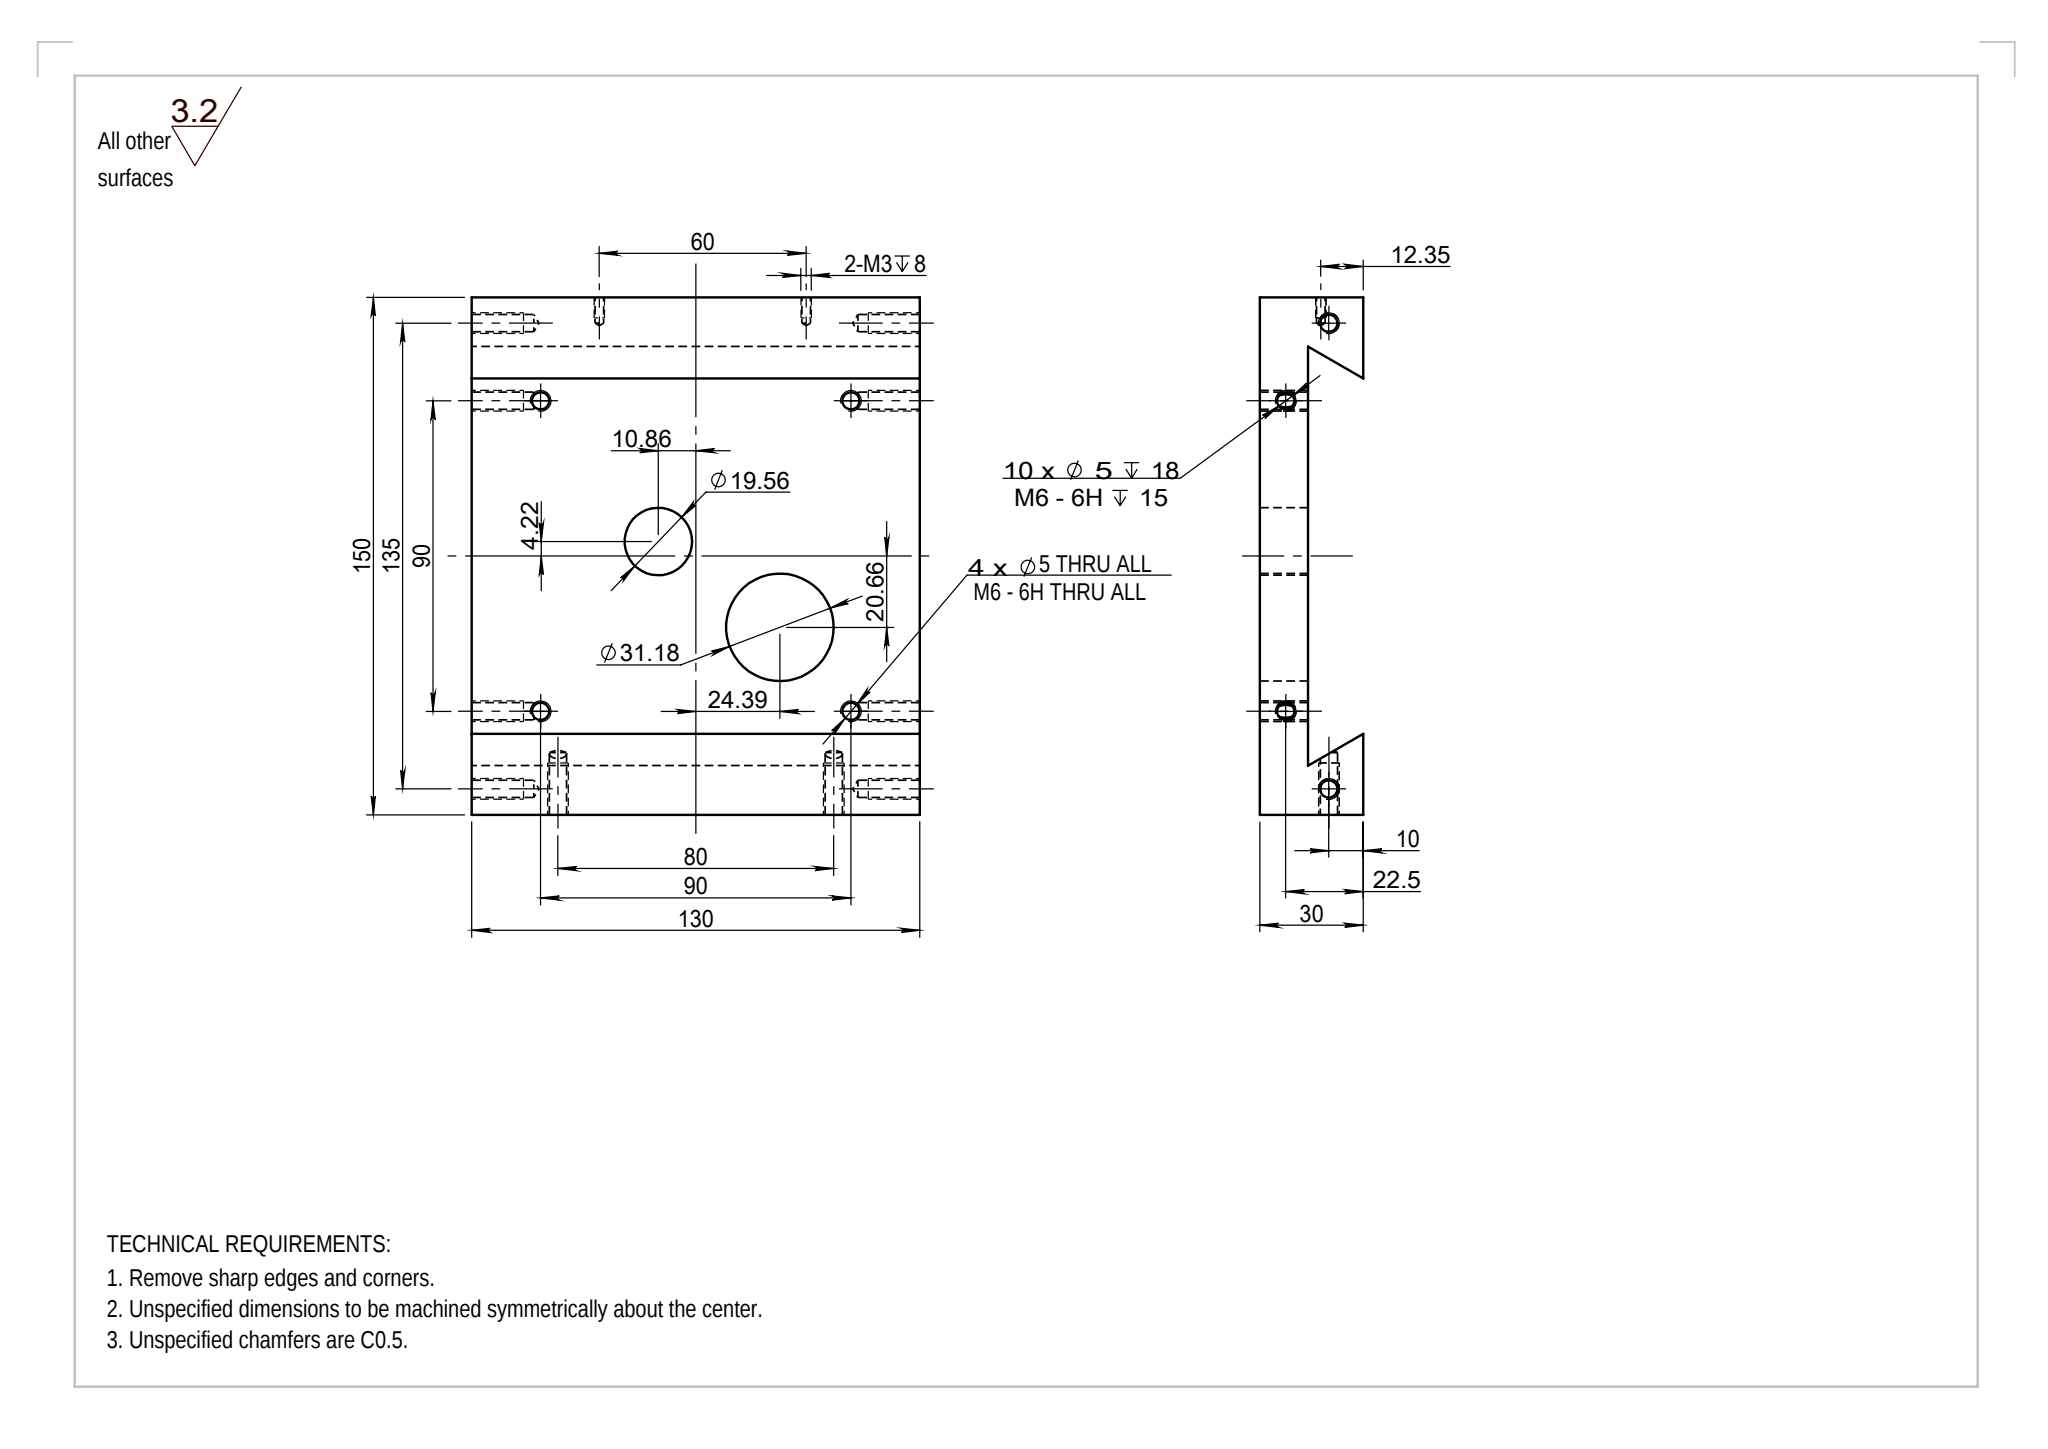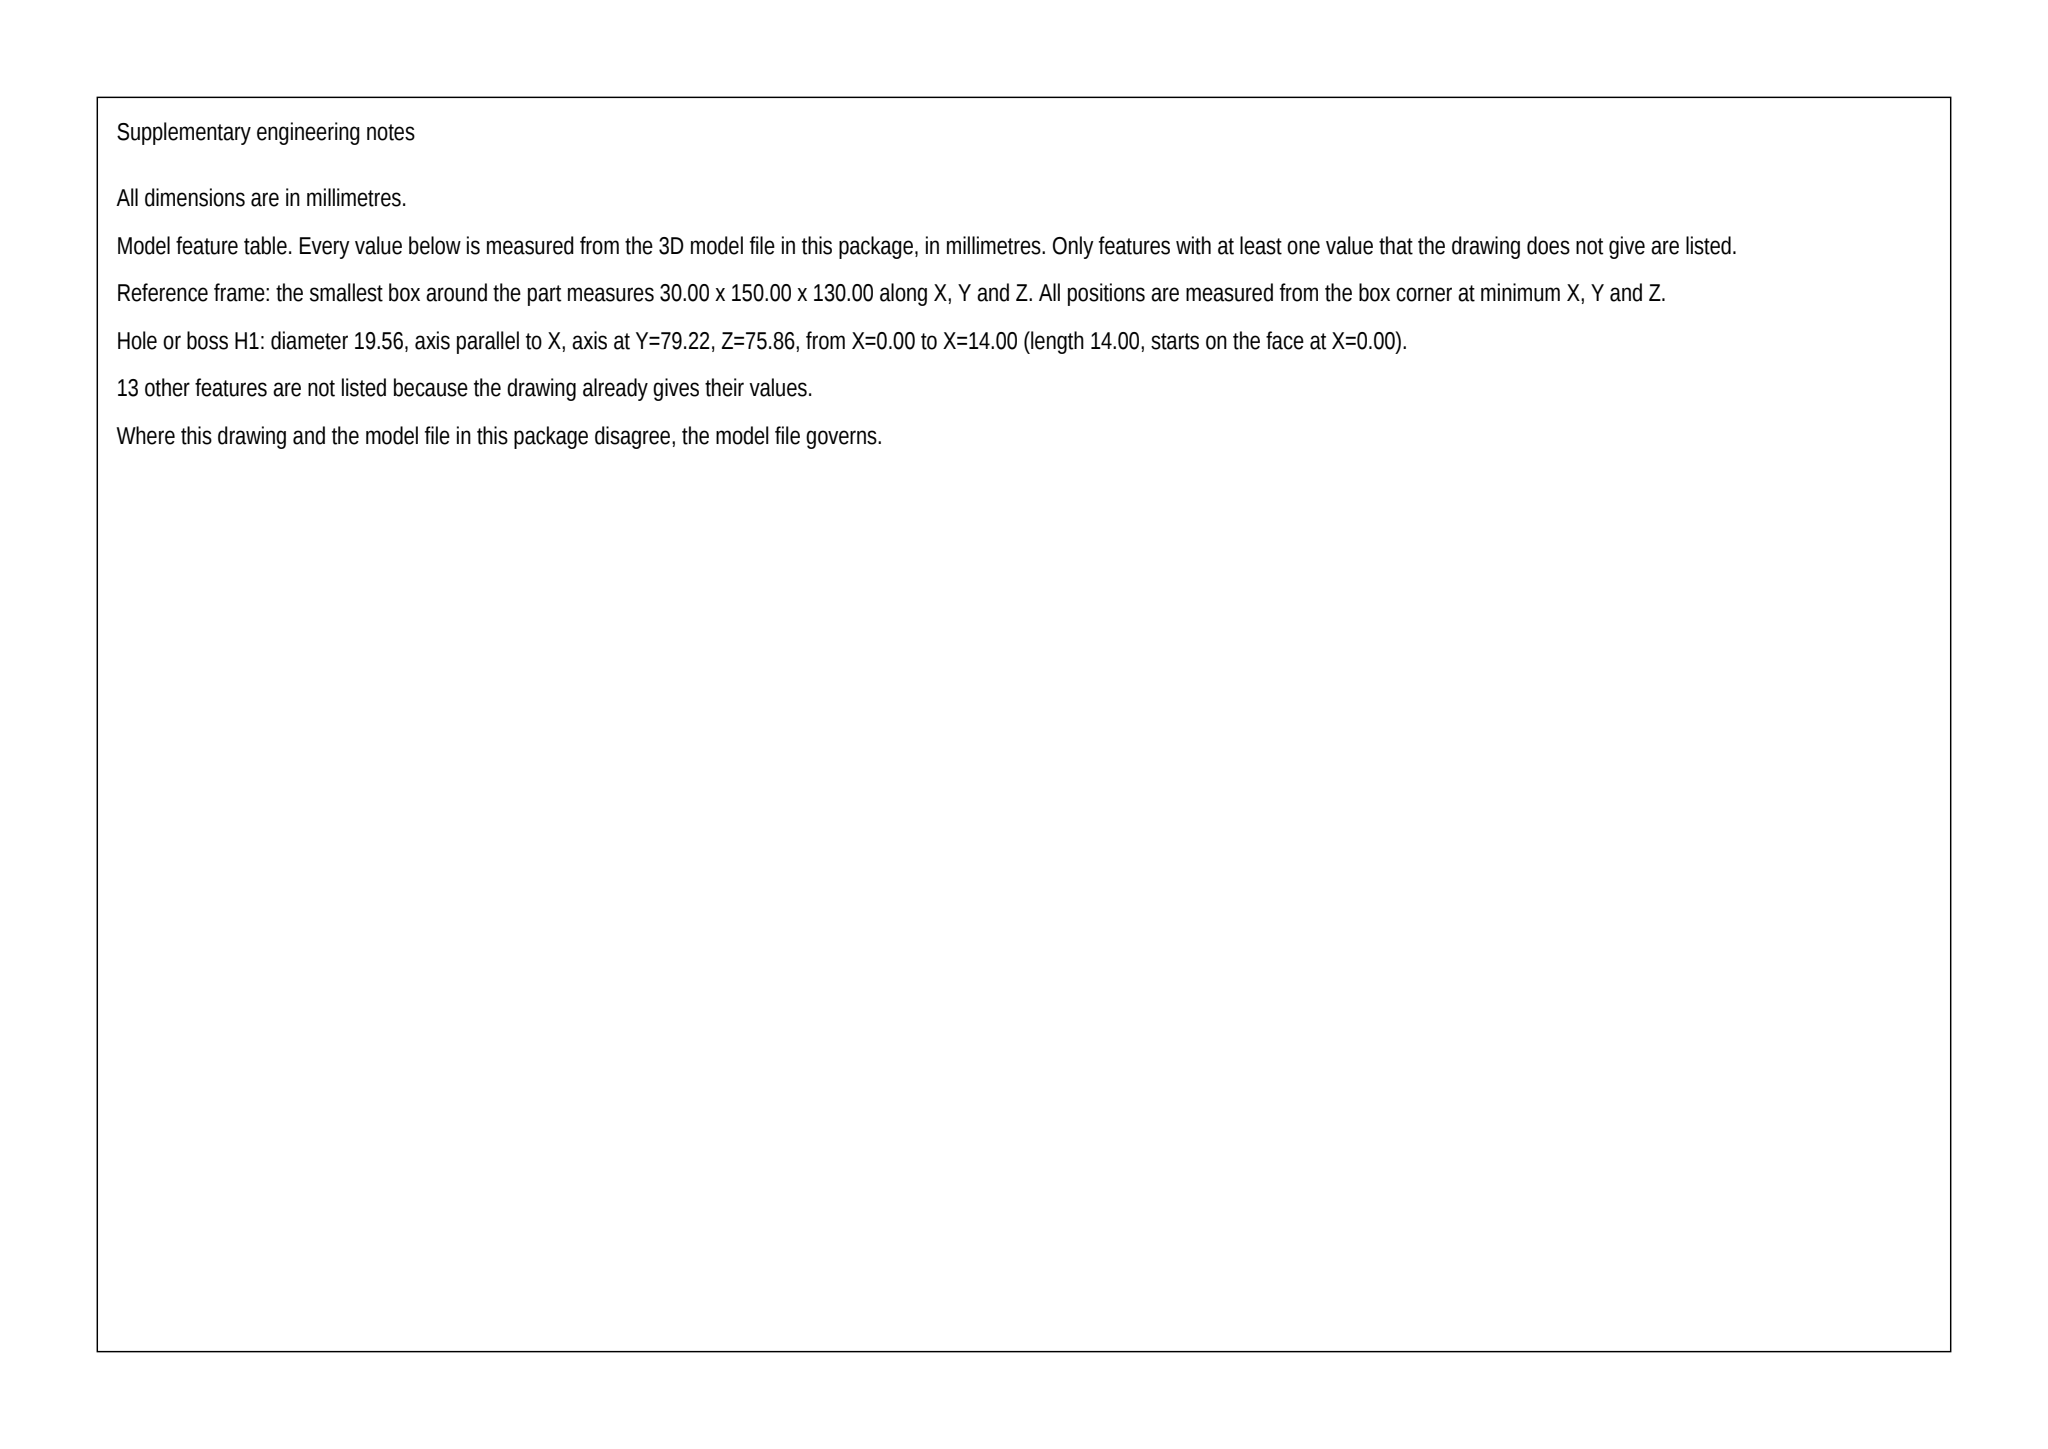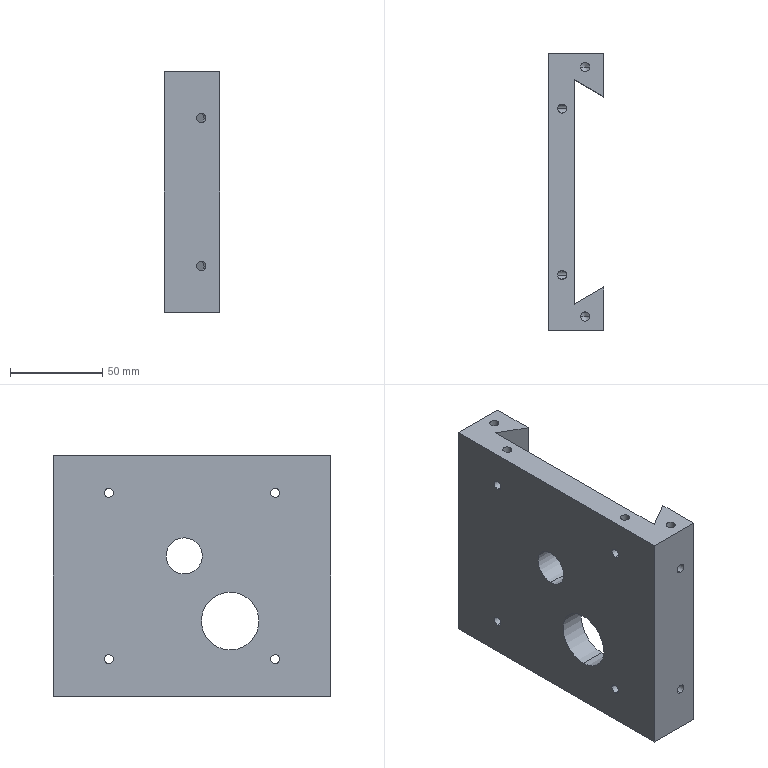Part | SolidWorks | mm | 1 solid | 68 faces | box 30 x 150 x 130 mm | volume 331934 mm3 | cylinder 36 | cone 22 | plane 10 | commonest cylinder face diameters 5 x28 2.5 x4 19.559 x2 31.176 x2
build123d program:
from build123d import *

# Parameters (mm, degrees)
BOSS_EXTRUDE1_DEPTH             = 130
M6_TAPPED_HOLE1_D               = 5
M6_TAPPED_HOLE1_DEPTH           = 18
M6_TAPPED_HOLE1_TIP             = 1.502
M6_TAPPED_HOLE1_ON_FACE_2_D     = 5
M6_TAPPED_HOLE1_ON_FACE_2_DEPTH = 18
M6_TAPPED_HOLE1_ON_FACE_2_TIP   = 1.502
M6_TAPPED_HOLE1_ON_FACE_3_D     = 5
M6_TAPPED_HOLE1_ON_FACE_3_DEPTH = 18
M6_TAPPED_HOLE1_ON_FACE_3_TIP   = 1.502
M6_TAPPED_HOLE3_D               = 5
M3_TAPPED_HOLE1_D               = 2.5
M3_TAPPED_HOLE1_DEPTH           = 7.5
M3_TAPPED_HOLE1_TIP             = 0.7511
SKETCH6_R                       = 9.779
SKETCH6_R_2                     = 15.588
CUT_EXTRUDE1_DEPTH              = 80


with BuildPart() as part:
    # Sketch1 → Boss-Extrude1 (new body)
    with BuildSketch(Plane.XY):
        Polygon((30, -75), (0, -75), (0, 75), (30, 75), (30, 51.5), (14, 60.738), (14, -60.738), (30, -51.5), align=None)
    extrude(amount=BOSS_EXTRUDE1_DEPTH)

    # M6 Tapped Hole1
    with Locations(Plane(origin=(7.5, 45, 130), x_dir=(1, 0, 0), z_dir=(0, 0, 1))):
        with Locations((0, 0), (0, -90), (12.5, -112.5), (12.5, 22.5)):
            Hole(M6_TAPPED_HOLE1_D / 2, depth=M6_TAPPED_HOLE1_DEPTH)
            with Locations((0, 0, -(M6_TAPPED_HOLE1_DEPTH + M6_TAPPED_HOLE1_TIP / 2))):  # 118° drill point
                Cone(0, M6_TAPPED_HOLE1_D / 2, M6_TAPPED_HOLE1_TIP, mode=Mode.SUBTRACT)

    # M6 Tapped Hole1 on face 2
    with Locations(Plane(origin=(20, 67.5, 0), x_dir=(-1, 0, 0), z_dir=(0, 0, -1))):
        with Locations((0, 0), (12.5, -22.5), (12.5, -112.5), (0, -135)):
            Hole(M6_TAPPED_HOLE1_ON_FACE_2_D / 2, depth=M6_TAPPED_HOLE1_ON_FACE_2_DEPTH)
            with Locations((0, 0, -(M6_TAPPED_HOLE1_ON_FACE_2_DEPTH + M6_TAPPED_HOLE1_ON_FACE_2_TIP / 2))):  # 118° drill point
                Cone(0, M6_TAPPED_HOLE1_ON_FACE_2_D / 2, M6_TAPPED_HOLE1_ON_FACE_2_TIP, mode=Mode.SUBTRACT)

    # M6 Tapped Hole1 on face 3
    with Locations(Plane(origin=(20, -75, 105), x_dir=(0, 0, -1), z_dir=(0, -1, 0))):
        with Locations((0, 0), (80, 0)):
            Hole(M6_TAPPED_HOLE1_ON_FACE_3_D / 2, depth=M6_TAPPED_HOLE1_ON_FACE_3_DEPTH)
            with Locations((0, 0, -(M6_TAPPED_HOLE1_ON_FACE_3_DEPTH + M6_TAPPED_HOLE1_ON_FACE_3_TIP / 2))):  # 118° drill point
                Cone(0, M6_TAPPED_HOLE1_ON_FACE_3_D / 2, M6_TAPPED_HOLE1_ON_FACE_3_TIP, mode=Mode.SUBTRACT)

    # M6 Tapped Hole3 (through all)
    with Locations(Plane(origin=(14, 45, 110), x_dir=(0, 0, 1), z_dir=(1, 0, 0))):
        with Locations((0, 0), (0, 90), (-90, 90), (-90, 0)):
            Hole(M6_TAPPED_HOLE3_D / 2)

    # M3 Tapped Hole1
    with Locations(Plane(origin=(0, 75, 0), x_dir=(1, 0, 0), z_dir=(0, 1, 0))):
        with Locations((17.648, -33), (17.648, -93)):
            Hole(M3_TAPPED_HOLE1_D / 2, depth=M3_TAPPED_HOLE1_DEPTH)
            with Locations((0, 0, -(M3_TAPPED_HOLE1_DEPTH + M3_TAPPED_HOLE1_TIP / 2))):  # 118° drill point
                Cone(0, M3_TAPPED_HOLE1_D / 2, M3_TAPPED_HOLE1_TIP, mode=Mode.SUBTRACT)

    # Sketch6 → Cut-Extrude1 (cut)
    with BuildSketch(Plane(origin=(14, 0, 0), x_dir=(0, 0, -1), z_dir=(1, 0, 0))):
        with Locations((-75.863, 4.218)):
            Circle(SKETCH6_R)
        with Locations((-40.607, -20.656)):
            Circle(SKETCH6_R_2)
    extrude(amount=-CUT_EXTRUDE1_DEPTH, mode=Mode.SUBTRACT)


solid = part.part